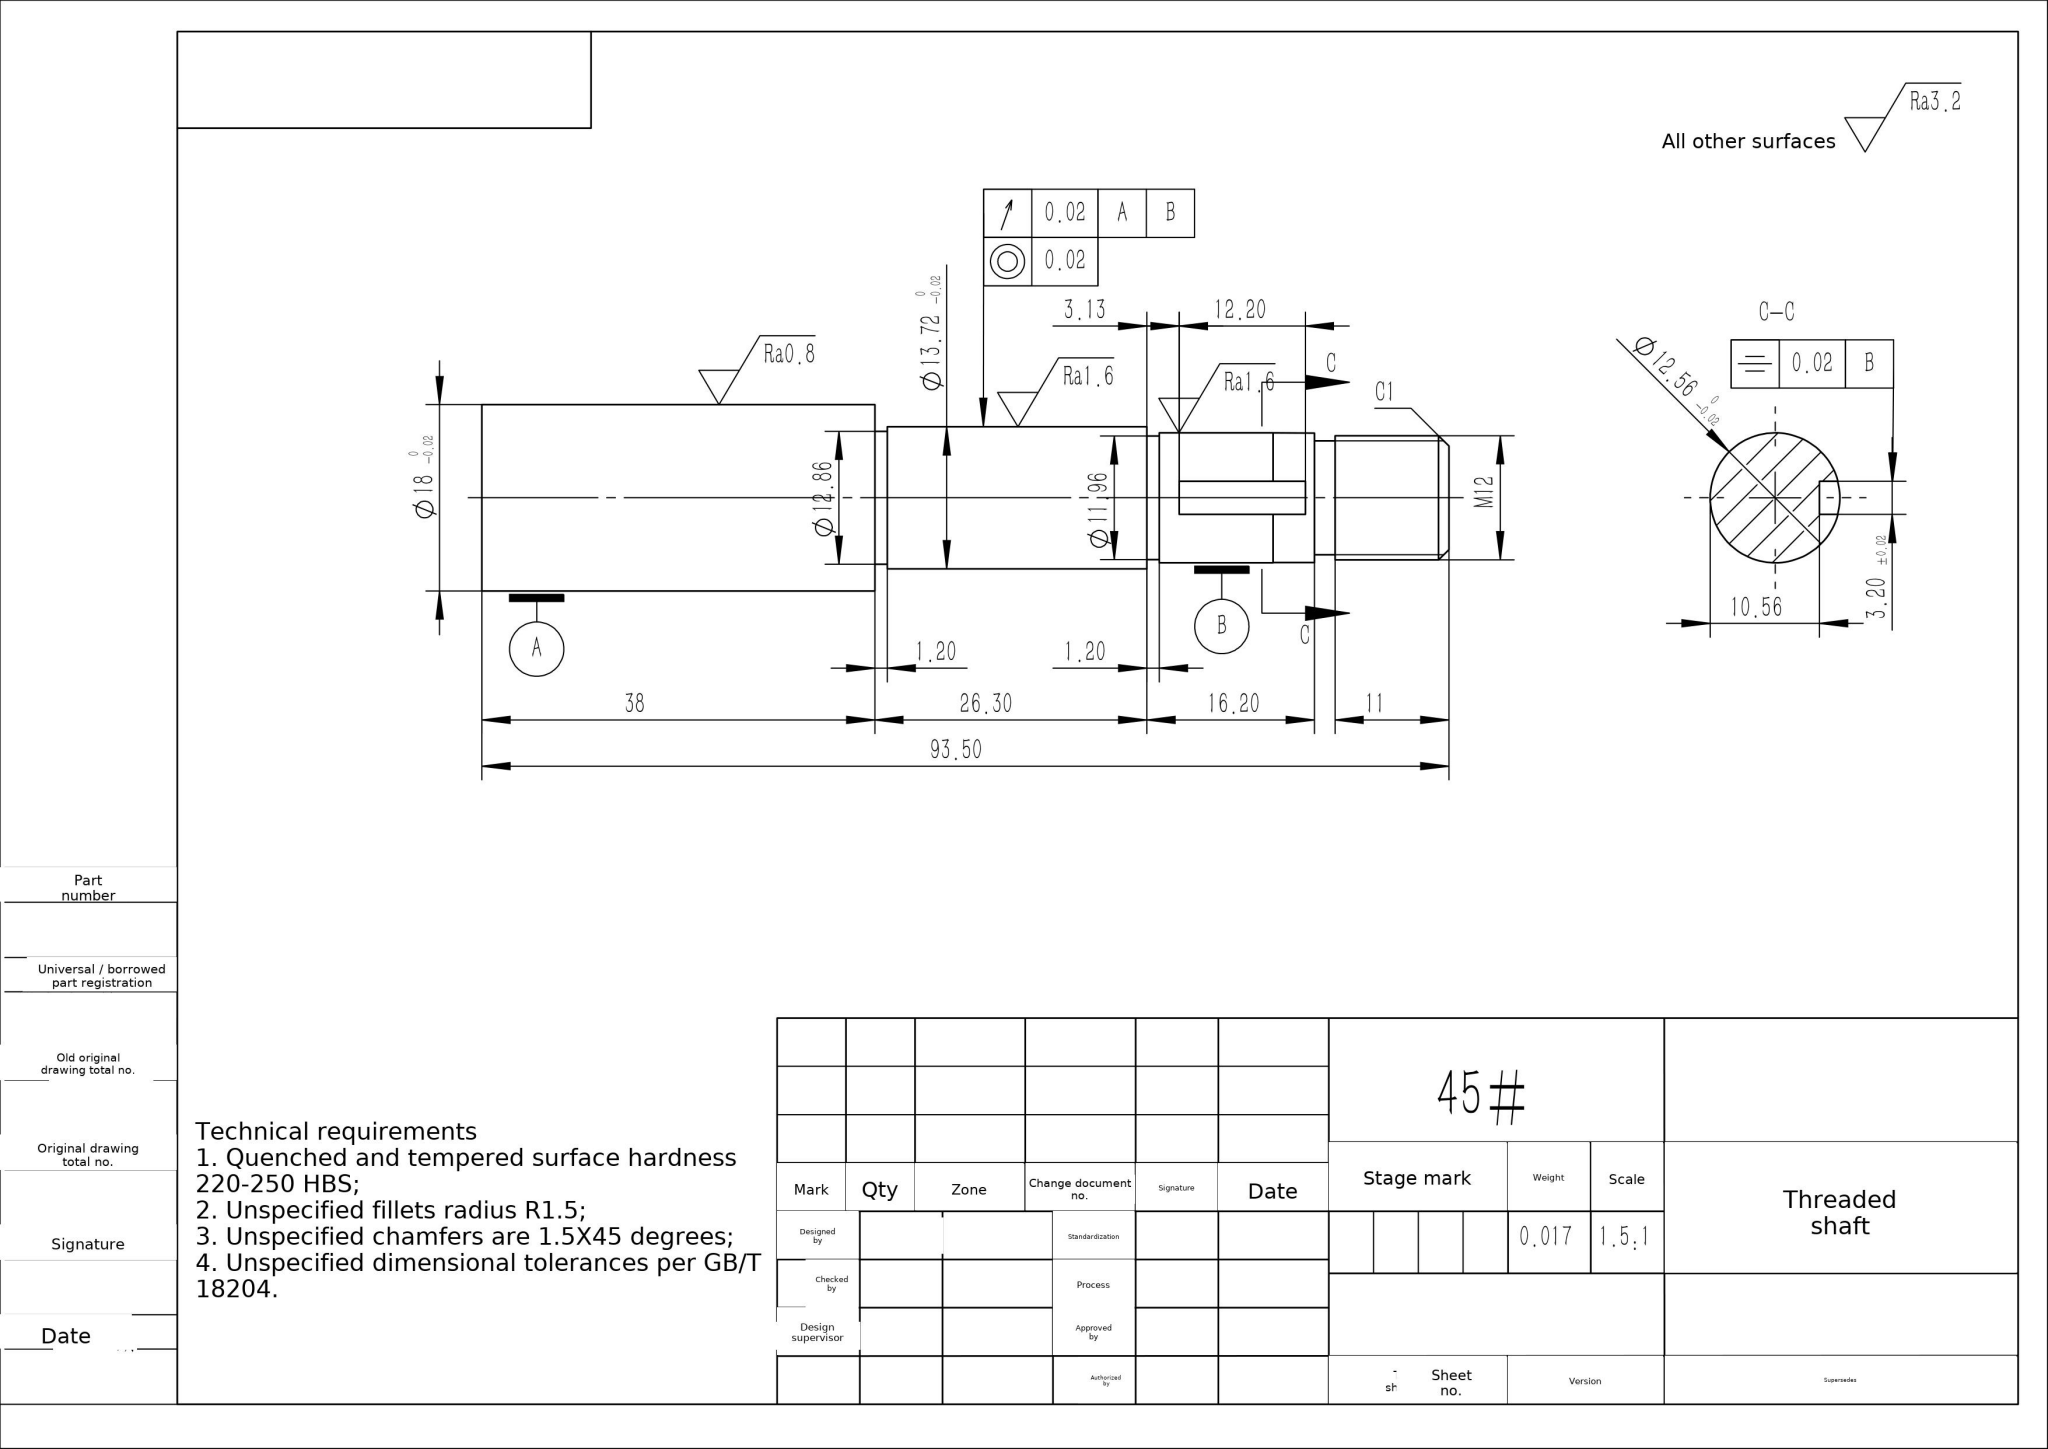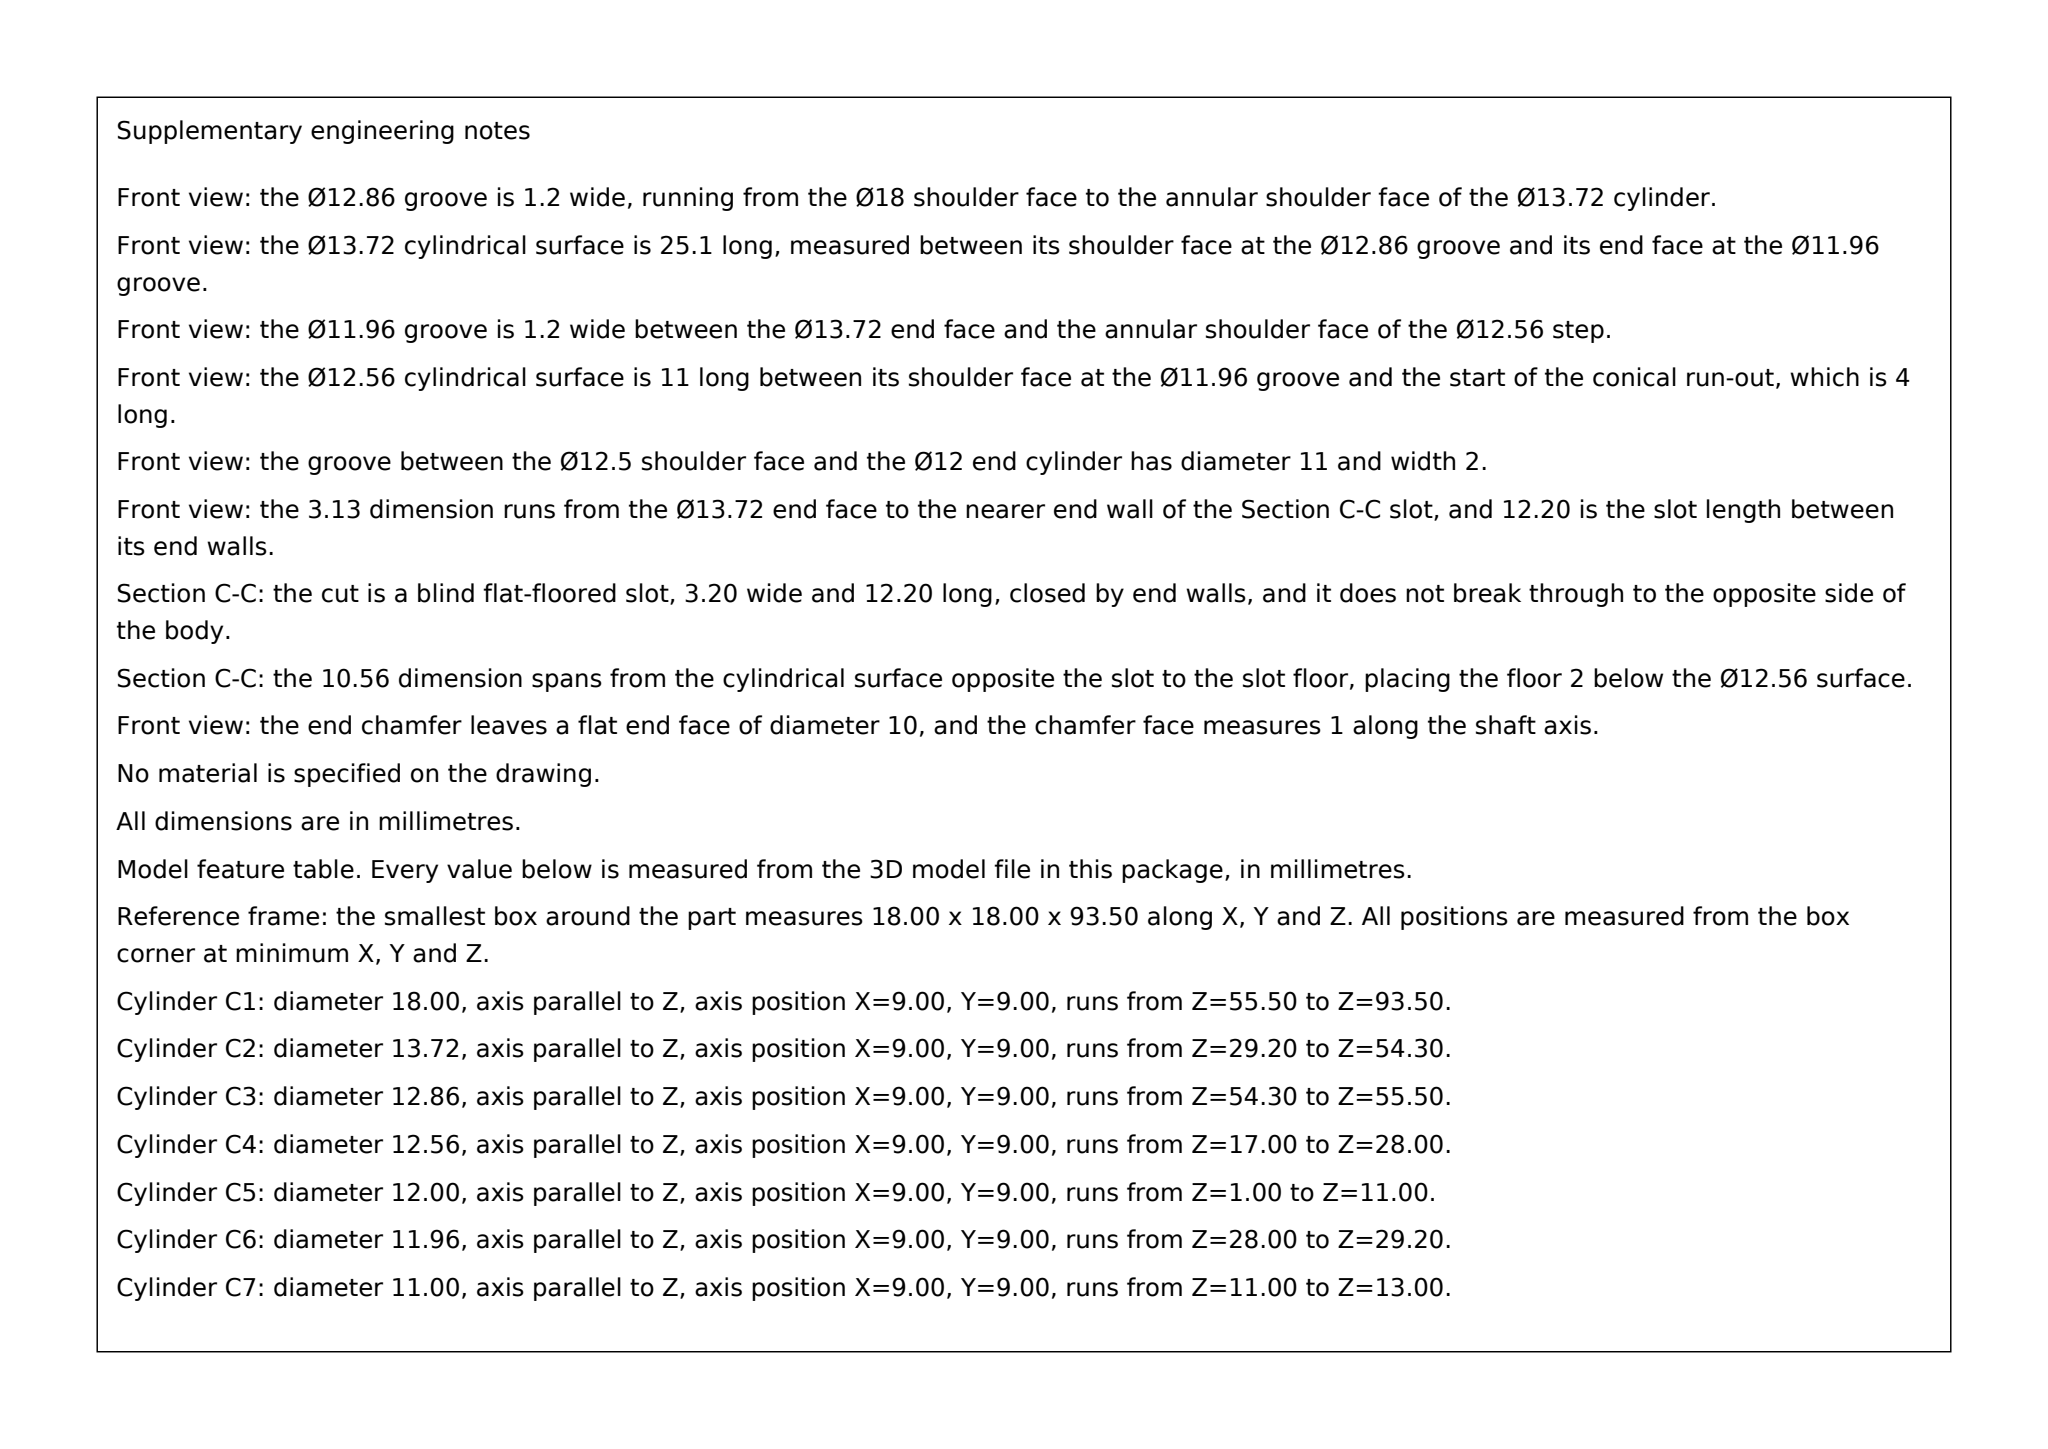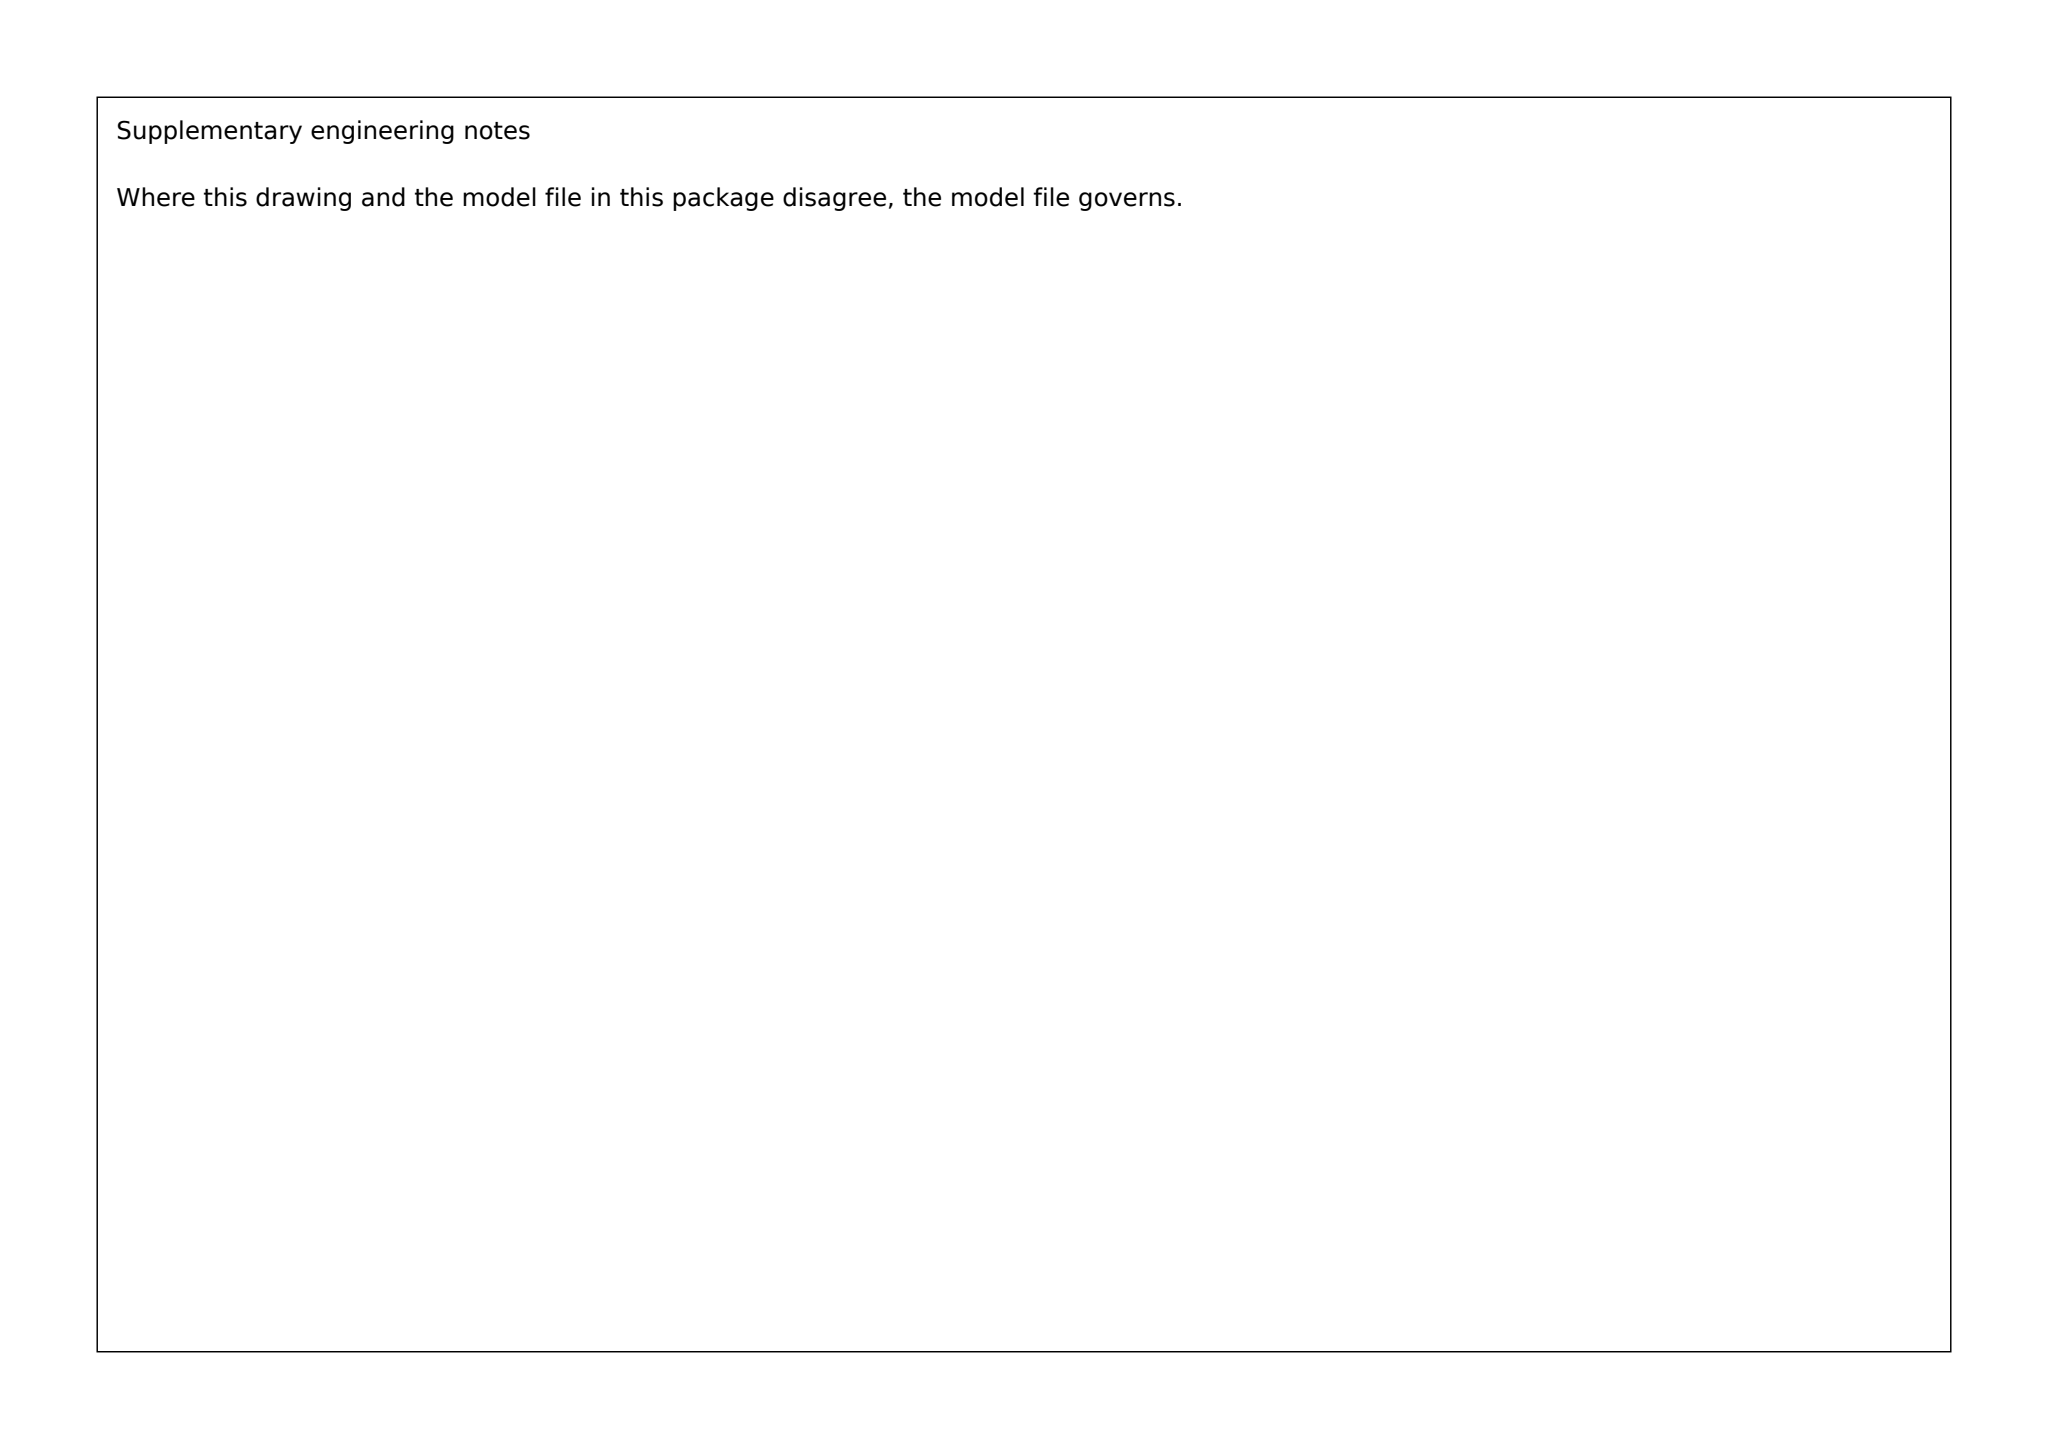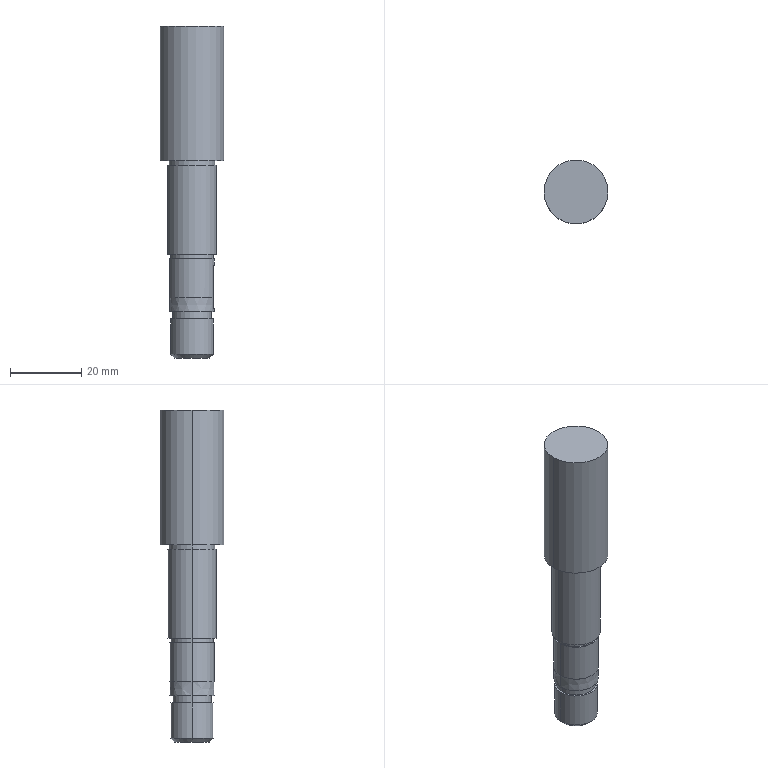Part | SolidWorks | mm | 1 solid | 32 faces | box 18 x 18 x 93.5 mm | volume 16868 mm3 | cylinder 14 | plane 14 | cone 4 | commonest cylinder face diameters 12 x2 11 x2 12.56 x2 11.96 x2 13.72 x2 12.86 x2 18 x2
Drawing notes:
THREAD RELIEF Ø11 x 2.0 WIDE BETWEEN Ø12.56 & M12 | from the solid: cylinder dia 11.0, axis z, length 2.0, spans z=11.0 to 13.0, between Ø12 thread (z=0-11) and Ø12.56 boss
RELIEF 2.0 LG, FROM 11 TO 13 OFF M12 THREAD END | from the solid: z planes at 11.0 and 13.0; 93.50 overall less 38+26.30+16.20+11 chain = 2.0 undimensioned segment
build123d program:
from build123d import *

# Parameters (mm, degrees)
SKETCH1_R           = 9
BOSS_EXTRUDE1_DEPTH = 38
SKETCH2_R           = 6.43
BOSS_EXTRUDE2_DEPTH = 1.2
SKETCH3_R           = 6.86
BOSS_EXTRUDE3_DEPTH = 25.1
SKETCH4_R           = 5.98
BOSS_EXTRUDE4_DEPTH = 1.2
SKETCH5_R           = 6.28
BOSS_EXTRUDE5_DEPTH = 11
SKETCH6_R           = 6.25
BOSS_EXTRUDE6_DEPTH = 4
SKETCH18_R          = 5.5
BOSS_EXTRUDE7_DEPTH = 2
SKETCH19_R          = 6
BOSS_EXTRUDE8_DEPTH = 11
SKETCH21_W          = 12.2
SKETCH21_H          = 3.2
CUT_EXTRUDE2_DEPTH  = 2
CHAMFER1_SIZE       = 1


with BuildPart() as part:
    # Sketch1 → Boss-Extrude1 (new body)
    with BuildSketch(Plane.XY):
        Circle(SKETCH1_R)
    extrude(amount=BOSS_EXTRUDE1_DEPTH)

    # Sketch2 → Boss-Extrude2 (add)
    with BuildSketch(Plane.XY):
        Circle(SKETCH2_R)
    extrude(amount=-BOSS_EXTRUDE2_DEPTH)

    # Sketch3 → Boss-Extrude3 (add)
    with BuildSketch(Plane(origin=(0, 0, -1.2), x_dir=(-1, 0, 0), z_dir=(0, 0, -1))):
        Circle(SKETCH3_R)
    extrude(amount=BOSS_EXTRUDE3_DEPTH)

    # Sketch4 → Boss-Extrude4 (add)
    with BuildSketch(Plane(origin=(0, 0, -26.3), x_dir=(-1, 0, 0), z_dir=(0, 0, -1))):
        Circle(SKETCH4_R)
    extrude(amount=BOSS_EXTRUDE4_DEPTH)

    # Sketch5 → Boss-Extrude5 (add)
    with BuildSketch(Plane(origin=(0, 0, -27.5), x_dir=(-1, 0, 0), z_dir=(0, 0, -1))):
        Circle(SKETCH5_R)
    extrude(amount=BOSS_EXTRUDE5_DEPTH)

    # Sketch6 → Boss-Extrude6 (add)
    with BuildSketch(Plane(origin=(0, 0, -38.5), x_dir=(-1, 0, 0), z_dir=(0, 0, -1))):
        Circle(SKETCH6_R)
    extrude(amount=BOSS_EXTRUDE6_DEPTH)

    # Sketch16 → Revolve1 (revolve)
    with BuildSketch(Plane(origin=(0, 0, 0), x_dir=(0, 0, -1), z_dir=(1, 0, 0)), mode=Mode.PRIVATE) as revolve1_sk:
        Polygon((38.5, 6.268), (38.5, 6.238), (42.5, 6.25), align=None)
    revolve(revolve1_sk.sketch.rotate(Axis((0, 0, -43.911), (0, 0, 1)), 90), axis=Axis((0, 0, -43.911), (0, 0, 1)))

    # Sketch18 → Boss-Extrude7 (add)
    with BuildSketch(Plane(origin=(0, 0, -42.5), x_dir=(-1, 0, 0), z_dir=(0, 0, -1))):
        Circle(SKETCH18_R)
    extrude(amount=BOSS_EXTRUDE7_DEPTH)

    # Sketch19 → Boss-Extrude8 (add)
    with BuildSketch(Plane(origin=(0, 0, -44.5), x_dir=(-1, 0, 0), z_dir=(0, 0, -1))):
        Circle(SKETCH19_R)
    extrude(amount=BOSS_EXTRUDE8_DEPTH)

    # Sketch21 → Cut-Extrude2 (cut)
    with BuildSketch(Plane(origin=(6.28, 0, 0), x_dir=(0, 0, -1), z_dir=(1, 0, 0))):
        with Locations((35.531, 0)):
            Rectangle(SKETCH21_W, SKETCH21_H)
    extrude(amount=-CUT_EXTRUDE2_DEPTH, mode=Mode.SUBTRACT)

    # Chamfer1
    chamfer1_edges = [part.edges().sort_by_distance(p)[0] for p in [
        (6, 0, -55.5),
    ]]
    chamfer(chamfer1_edges, length=CHAMFER1_SIZE)


solid = part.part